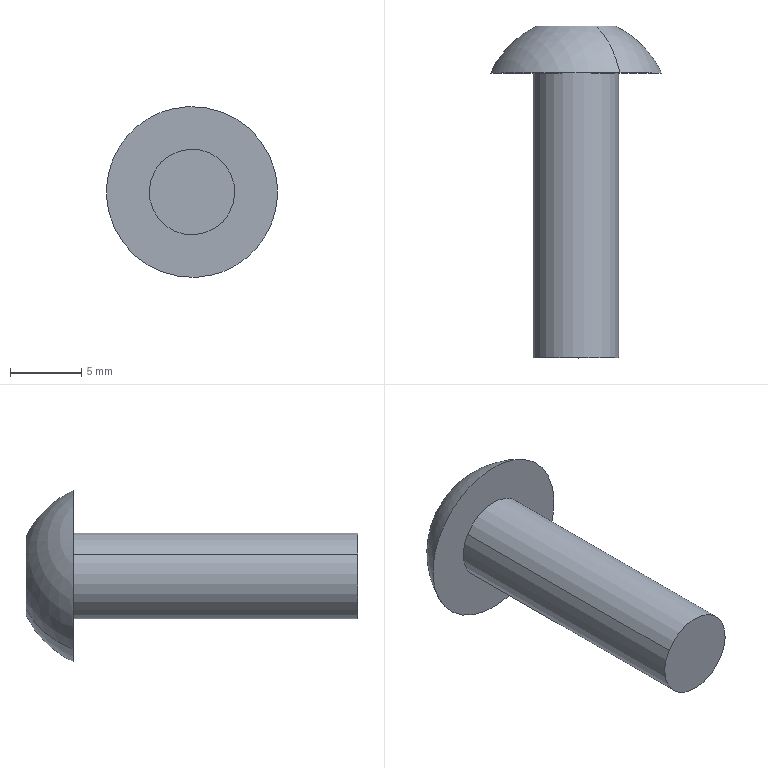Component | SolidWorks | RR40-1_hexagon socket button head screws gb-2 | 1 solid | 19 faces | box 12 x 23.3 x 12 mm | volume 776 mm3 | plane 15 | sphere 2 | cylinder 2 | commonest cylinder face diameters 6 x2
STEP:
#1=COLOUR_RGB('',0.7922,0.8196,0.9333);
#2=FILL_AREA_STYLE_COLOUR('',#1);
#3=FILL_AREA_STYLE('',(#2));
#4=SURFACE_STYLE_FILL_AREA(#3);
#5=SURFACE_SIDE_STYLE('',(#4));
#6=SURFACE_STYLE_USAGE(.BOTH.,#5);
#7=PRESENTATION_STYLE_ASSIGNMENT((#6));
#8=CARTESIAN_POINT('',(23.147,37.717,-81.266));
#9=VERTEX_POINT('',#8);
#10=CARTESIAN_POINT('',(23.39,37.717,-80.861));
#11=VERTEX_POINT('',#10);
#12=CARTESIAN_POINT('',(23.268,37.717,-81.063));
#13=DIRECTION('',(0.,1.,-0.));
#14=DIRECTION('',(0.8574,0.,-0.5146));
#15=AXIS2_PLACEMENT_3D('',#12,#13,#14);
#16=CIRCLE('',#15,0.2362);
#17=EDGE_CURVE('',#9,#11,#16,.T.);
#18=ORIENTED_EDGE('',*,*,#17,.T.);
#19=CARTESIAN_POINT('',(23.324,37.846,-80.97));
#20=VERTEX_POINT('',#19);
#21=CARTESIAN_POINT('',(23.268,37.612,-81.063));
#22=DIRECTION('',(-0.8574,0.,0.5146));
#23=DIRECTION('',(0.5146,0.,0.8574));
#24=AXIS2_PLACEMENT_3D('',#21,#22,#23);
#25=CIRCLE('',#24,0.2584);
#26=EDGE_CURVE('',#11,#20,#25,.T.);
#27=ORIENTED_EDGE('',*,*,#26,.T.);
#28=CARTESIAN_POINT('',(23.213,37.846,-81.156));
#29=VERTEX_POINT('',#28);
#30=CARTESIAN_POINT('',(23.268,37.846,-81.063));
#31=DIRECTION('',(0.,1.,-0.));
#32=DIRECTION('',(0.8574,0.,-0.5146));
#33=AXIS2_PLACEMENT_3D('',#30,#31,#32);
#34=CIRCLE('',#33,0.1083);
#35=EDGE_CURVE('',#29,#20,#34,.T.);
#36=ORIENTED_EDGE('',*,*,#35,.F.);
#37=CARTESIAN_POINT('',(23.268,37.612,-81.063));
#38=DIRECTION('',(0.8574,-0.,-0.5146));
#39=DIRECTION('',(-0.5146,0.,-0.8574));
#40=AXIS2_PLACEMENT_3D('',#37,#38,#39);
#41=CIRCLE('',#40,0.2584);
#42=EDGE_CURVE('',#9,#29,#41,.T.);
#43=ORIENTED_EDGE('',*,*,#42,.F.);
#44=EDGE_LOOP('',(#18,#27,#36,#43));
#45=FACE_OUTER_BOUND('',#44,.T.);
#46=CARTESIAN_POINT('',(23.268,37.612,-81.063));
#47=DIRECTION('',(-0.8574,0.,0.5146));
#48=DIRECTION('',(-0.5146,0.,-0.8574));
#49=AXIS2_PLACEMENT_3D('',#46,#47,#48);
#50=SPHERICAL_SURFACE('',#49,0.2584);
#51=ADVANCED_FACE('',(#45),#50,.T.);
#52=CARTESIAN_POINT('',(23.167,36.929,-81.002));
#53=VERTEX_POINT('',#52);
#54=CARTESIAN_POINT('',(23.37,36.929,-81.124));
#55=VERTEX_POINT('',#54);
#56=CARTESIAN_POINT('',(23.268,36.929,-81.063));
#57=DIRECTION('',(-0.,-1.,0.));
#58=DIRECTION('',(-0.8574,0.,0.5146));
#59=AXIS2_PLACEMENT_3D('',#56,#57,#58);
#60=CIRCLE('',#59,0.1181);
#61=EDGE_CURVE('',#53,#55,#60,.T.);
#62=ORIENTED_EDGE('',*,*,#61,.F.);
#63=CARTESIAN_POINT('',(23.167,37.717,-81.002));
#64=VERTEX_POINT('',#63);
#65=CARTESIAN_POINT('',(23.167,36.929,-81.002));
#66=DIRECTION('',(0.,1.,-0.));
#67=VECTOR('',#66,39.37);
#68=LINE('',#65,#67);
#69=EDGE_CURVE('',#53,#64,#68,.T.);
#70=ORIENTED_EDGE('',*,*,#69,.T.);
#71=CARTESIAN_POINT('',(23.37,37.717,-81.124));
#72=VERTEX_POINT('',#71);
#73=CARTESIAN_POINT('',(23.268,37.717,-81.063));
#74=DIRECTION('',(-0.,-1.,0.));
#75=DIRECTION('',(-0.8574,0.,0.5146));
#76=AXIS2_PLACEMENT_3D('',#73,#74,#75);
#77=CIRCLE('',#76,0.1181);
#78=EDGE_CURVE('',#64,#72,#77,.T.);
#79=ORIENTED_EDGE('',*,*,#78,.T.);
#80=CARTESIAN_POINT('',(23.37,36.929,-81.124));
#81=DIRECTION('',(0.,1.,-0.));
#82=VECTOR('',#81,39.37);
#83=LINE('',#80,#82);
#84=EDGE_CURVE('',#55,#72,#83,.T.);
#85=ORIENTED_EDGE('',*,*,#84,.F.);
#86=EDGE_LOOP('',(#62,#70,#79,#85));
#87=FACE_OUTER_BOUND('',#86,.T.);
#88=CARTESIAN_POINT('',(23.268,36.929,-81.063));
#89=DIRECTION('',(0.,1.,-0.));
#90=DIRECTION('',(0.8574,0.,-0.5146));
#91=AXIS2_PLACEMENT_3D('',#88,#89,#90);
#92=CYLINDRICAL_SURFACE('',#91,0.1181);
#93=ADVANCED_FACE('',(#87),#92,.T.);
#94=ORIENTED_EDGE('',*,*,#35,.T.);
#95=CARTESIAN_POINT('',(23.268,37.846,-81.063));
#96=DIRECTION('',(0.,1.,-0.));
#97=DIRECTION('',(0.8574,0.,-0.5146));
#98=AXIS2_PLACEMENT_3D('',#95,#96,#97);
#99=CIRCLE('',#98,0.1083);
#100=EDGE_CURVE('',#20,#29,#99,.T.);
#101=ORIENTED_EDGE('',*,*,#100,.T.);
#102=EDGE_LOOP('',(#94,#101));
#103=FACE_OUTER_BOUND('',#102,.T.);
#104=CARTESIAN_POINT('',(23.27,37.846,-80.972));
#105=VERTEX_POINT('',#104);
#106=CARTESIAN_POINT('',(23.19,37.846,-81.016));
#107=VERTEX_POINT('',#106);
#108=CARTESIAN_POINT('',(23.27,37.846,-80.972));
#109=DIRECTION('',(-0.8744,0.,-0.4852));
#110=VECTOR('',#109,39.37);
#111=LINE('',#108,#110);
#112=EDGE_CURVE('',#105,#107,#111,.T.);
#113=ORIENTED_EDGE('',*,*,#112,.T.);
#114=CARTESIAN_POINT('',(23.189,37.846,-81.107));
#115=VERTEX_POINT('',#114);
#116=CARTESIAN_POINT('',(23.19,37.846,-81.016));
#117=DIRECTION('',(-0.01698,-0.,-0.9999));
#118=VECTOR('',#117,39.37);
#119=LINE('',#116,#118);
#120=EDGE_CURVE('',#107,#115,#119,.T.);
#121=ORIENTED_EDGE('',*,*,#120,.T.);
#122=CARTESIAN_POINT('',(23.267,37.846,-81.154));
#123=VERTEX_POINT('',#122);
#124=CARTESIAN_POINT('',(23.189,37.846,-81.107));
#125=DIRECTION('',(0.8574,-0.,-0.5146));
#126=VECTOR('',#125,39.37);
#127=LINE('',#124,#126);
#128=EDGE_CURVE('',#115,#123,#127,.T.);
#129=ORIENTED_EDGE('',*,*,#128,.T.);
#130=CARTESIAN_POINT('',(23.346,37.846,-81.11));
#131=VERTEX_POINT('',#130);
#132=CARTESIAN_POINT('',(23.267,37.846,-81.154));
#133=DIRECTION('',(0.8744,-0.,0.4852));
#134=VECTOR('',#133,39.37);
#135=LINE('',#132,#134);
#136=EDGE_CURVE('',#123,#131,#135,.T.);
#137=ORIENTED_EDGE('',*,*,#136,.T.);
#138=CARTESIAN_POINT('',(23.348,37.846,-81.019));
#139=VERTEX_POINT('',#138);
#140=CARTESIAN_POINT('',(23.346,37.846,-81.11));
#141=DIRECTION('',(0.01698,0.,0.9999));
#142=VECTOR('',#141,39.37);
#143=LINE('',#140,#142);
#144=EDGE_CURVE('',#131,#139,#143,.T.);
#145=ORIENTED_EDGE('',*,*,#144,.T.);
#146=CARTESIAN_POINT('',(23.348,37.846,-81.019));
#147=DIRECTION('',(-0.8574,0.,0.5146));
#148=VECTOR('',#147,39.37);
#149=LINE('',#146,#148);
#150=EDGE_CURVE('',#139,#105,#149,.T.);
#151=ORIENTED_EDGE('',*,*,#150,.T.);
#152=EDGE_LOOP('',(#113,#121,#129,#137,#145,#151));
#153=FACE_BOUND('',#152,.T.);
#154=CARTESIAN_POINT('',(23.268,37.846,-81.063));
#155=DIRECTION('',(-0.,-1.,0.));
#156=DIRECTION('',(-0.8574,0.,0.5146));
#157=AXIS2_PLACEMENT_3D('',#154,#155,#156);
#158=PLANE('',#157);
#159=ADVANCED_FACE('',(#103,#153),#158,.F.);
#160=ORIENTED_EDGE('',*,*,#17,.F.);
#161=CARTESIAN_POINT('',(23.268,37.717,-81.063));
#162=DIRECTION('',(0.,1.,-0.));
#163=DIRECTION('',(0.8574,0.,-0.5146));
#164=AXIS2_PLACEMENT_3D('',#161,#162,#163);
#165=CIRCLE('',#164,0.2362);
#166=EDGE_CURVE('',#11,#9,#165,.T.);
#167=ORIENTED_EDGE('',*,*,#166,.F.);
#168=EDGE_LOOP('',(#160,#167));
#169=FACE_OUTER_BOUND('',#168,.T.);
#170=CARTESIAN_POINT('',(23.268,37.717,-81.063));
#171=DIRECTION('',(-0.,-1.,0.));
#172=DIRECTION('',(-0.8574,0.,0.5146));
#173=AXIS2_PLACEMENT_3D('',#170,#171,#172);
#174=CIRCLE('',#173,0.1181);
#175=EDGE_CURVE('',#72,#64,#174,.T.);
#176=ORIENTED_EDGE('',*,*,#175,.F.);
#177=ORIENTED_EDGE('',*,*,#78,.F.);
#178=EDGE_LOOP('',(#176,#177));
#179=FACE_BOUND('',#178,.T.);
#180=CARTESIAN_POINT('',(23.268,37.717,-81.063));
#181=DIRECTION('',(-0.,-1.,0.));
#182=DIRECTION('',(-0.8574,0.,0.5146));
#183=AXIS2_PLACEMENT_3D('',#180,#181,#182);
#184=PLANE('',#183);
#185=ADVANCED_FACE('',(#169,#179),#184,.T.);
#186=ORIENTED_EDGE('',*,*,#69,.F.);
#187=CARTESIAN_POINT('',(23.268,36.929,-81.063));
#188=DIRECTION('',(-0.,-1.,0.));
#189=DIRECTION('',(-0.8574,0.,0.5146));
#190=AXIS2_PLACEMENT_3D('',#187,#188,#189);
#191=CIRCLE('',#190,0.1181);
#192=EDGE_CURVE('',#55,#53,#191,.T.);
#193=ORIENTED_EDGE('',*,*,#192,.F.);
#194=ORIENTED_EDGE('',*,*,#84,.T.);
#195=ORIENTED_EDGE('',*,*,#175,.T.);
#196=EDGE_LOOP('',(#186,#193,#194,#195));
#197=FACE_OUTER_BOUND('',#196,.T.);
#198=CARTESIAN_POINT('',(23.268,36.929,-81.063));
#199=DIRECTION('',(0.,1.,-0.));
#200=DIRECTION('',(0.8574,0.,-0.5146));
#201=AXIS2_PLACEMENT_3D('',#198,#199,#200);
#202=CYLINDRICAL_SURFACE('',#201,0.1181);
#203=ADVANCED_FACE('',(#197),#202,.T.);
#204=ORIENTED_EDGE('',*,*,#192,.T.);
#205=ORIENTED_EDGE('',*,*,#61,.T.);
#206=EDGE_LOOP('',(#204,#205));
#207=FACE_OUTER_BOUND('',#206,.T.);
#208=CARTESIAN_POINT('',(23.268,36.929,-81.063));
#209=DIRECTION('',(-0.,-1.,0.));
#210=DIRECTION('',(-0.8574,0.,0.5146));
#211=AXIS2_PLACEMENT_3D('',#208,#209,#210);
#212=PLANE('',#211);
#213=ADVANCED_FACE('',(#207),#212,.T.);
#214=ORIENTED_EDGE('',*,*,#26,.F.);
#215=ORIENTED_EDGE('',*,*,#166,.T.);
#216=ORIENTED_EDGE('',*,*,#42,.T.);
#217=ORIENTED_EDGE('',*,*,#100,.F.);
#218=EDGE_LOOP('',(#214,#215,#216,#217));
#219=FACE_OUTER_BOUND('',#218,.T.);
#220=CARTESIAN_POINT('',(23.268,37.612,-81.063));
#221=DIRECTION('',(-0.8574,0.,0.5146));
#222=DIRECTION('',(-0.5146,0.,-0.8574));
#223=AXIS2_PLACEMENT_3D('',#220,#221,#222);
#224=SPHERICAL_SURFACE('',#223,0.2584);
#225=ADVANCED_FACE('',(#219),#224,.T.);
#226=ORIENTED_EDGE('',*,*,#112,.F.);
#227=CARTESIAN_POINT('',(23.27,37.765,-80.972));
#228=VERTEX_POINT('',#227);
#229=CARTESIAN_POINT('',(23.27,37.765,-80.972));
#230=DIRECTION('',(0.,1.,-0.));
#231=VECTOR('',#230,39.37);
#232=LINE('',#229,#231);
#233=EDGE_CURVE('',#228,#105,#232,.T.);
#234=ORIENTED_EDGE('',*,*,#233,.F.);
#235=CARTESIAN_POINT('',(23.19,37.765,-81.016));
#236=VERTEX_POINT('',#235);
#237=CARTESIAN_POINT('',(23.27,37.765,-80.972));
#238=DIRECTION('',(-0.8744,0.,-0.4852));
#239=VECTOR('',#238,39.37);
#240=LINE('',#237,#239);
#241=EDGE_CURVE('',#228,#236,#240,.T.);
#242=ORIENTED_EDGE('',*,*,#241,.T.);
#243=CARTESIAN_POINT('',(23.19,37.765,-81.016));
#244=DIRECTION('',(0.,1.,-0.));
#245=VECTOR('',#244,39.37);
#246=LINE('',#243,#245);
#247=EDGE_CURVE('',#236,#107,#246,.T.);
#248=ORIENTED_EDGE('',*,*,#247,.T.);
#249=EDGE_LOOP('',(#226,#234,#242,#248));
#250=FACE_OUTER_BOUND('',#249,.T.);
#251=CARTESIAN_POINT('',(23.27,37.765,-80.972));
#252=DIRECTION('',(0.4852,-0.,-0.8744));
#253=DIRECTION('',(0.8744,-0.,0.4852));
#254=AXIS2_PLACEMENT_3D('',#251,#252,#253);
#255=PLANE('',#254);
#256=ADVANCED_FACE('',(#250),#255,.T.);
#257=ORIENTED_EDGE('',*,*,#120,.F.);
#258=ORIENTED_EDGE('',*,*,#247,.F.);
#259=CARTESIAN_POINT('',(23.189,37.765,-81.107));
#260=VERTEX_POINT('',#259);
#261=CARTESIAN_POINT('',(23.19,37.765,-81.016));
#262=DIRECTION('',(-0.01698,-0.,-0.9999));
#263=VECTOR('',#262,39.37);
#264=LINE('',#261,#263);
#265=EDGE_CURVE('',#236,#260,#264,.T.);
#266=ORIENTED_EDGE('',*,*,#265,.T.);
#267=CARTESIAN_POINT('',(23.189,37.765,-81.107));
#268=DIRECTION('',(0.,1.,-0.));
#269=VECTOR('',#268,39.37);
#270=LINE('',#267,#269);
#271=EDGE_CURVE('',#260,#115,#270,.T.);
#272=ORIENTED_EDGE('',*,*,#271,.T.);
#273=EDGE_LOOP('',(#257,#258,#266,#272));
#274=FACE_OUTER_BOUND('',#273,.T.);
#275=CARTESIAN_POINT('',(23.19,37.765,-81.016));
#276=DIRECTION('',(0.9999,-0.,-0.01698));
#277=DIRECTION('',(0.01698,0.,0.9999));
#278=AXIS2_PLACEMENT_3D('',#275,#276,#277);
#279=PLANE('',#278);
#280=ADVANCED_FACE('',(#274),#279,.T.);
#281=ORIENTED_EDGE('',*,*,#128,.F.);
#282=ORIENTED_EDGE('',*,*,#271,.F.);
#283=CARTESIAN_POINT('',(23.267,37.765,-81.154));
#284=VERTEX_POINT('',#283);
#285=CARTESIAN_POINT('',(23.189,37.765,-81.107));
#286=DIRECTION('',(0.8574,-0.,-0.5146));
#287=VECTOR('',#286,39.37);
#288=LINE('',#285,#287);
#289=EDGE_CURVE('',#260,#284,#288,.T.);
#290=ORIENTED_EDGE('',*,*,#289,.T.);
#291=CARTESIAN_POINT('',(23.267,37.765,-81.154));
#292=DIRECTION('',(0.,1.,-0.));
#293=VECTOR('',#292,39.37);
#294=LINE('',#291,#293);
#295=EDGE_CURVE('',#284,#123,#294,.T.);
#296=ORIENTED_EDGE('',*,*,#295,.T.);
#297=EDGE_LOOP('',(#281,#282,#290,#296));
#298=FACE_OUTER_BOUND('',#297,.T.);
#299=CARTESIAN_POINT('',(23.189,37.765,-81.107));
#300=DIRECTION('',(0.5146,-0.,0.8574));
#301=DIRECTION('',(-0.8574,0.,0.5146));
#302=AXIS2_PLACEMENT_3D('',#299,#300,#301);
#303=PLANE('',#302);
#304=ADVANCED_FACE('',(#298),#303,.T.);
#305=ORIENTED_EDGE('',*,*,#136,.F.);
#306=ORIENTED_EDGE('',*,*,#295,.F.);
#307=CARTESIAN_POINT('',(23.346,37.765,-81.11));
#308=VERTEX_POINT('',#307);
#309=CARTESIAN_POINT('',(23.267,37.765,-81.154));
#310=DIRECTION('',(0.8744,-0.,0.4852));
#311=VECTOR('',#310,39.37);
#312=LINE('',#309,#311);
#313=EDGE_CURVE('',#284,#308,#312,.T.);
#314=ORIENTED_EDGE('',*,*,#313,.T.);
#315=CARTESIAN_POINT('',(23.346,37.765,-81.11));
#316=DIRECTION('',(0.,1.,-0.));
#317=VECTOR('',#316,39.37);
#318=LINE('',#315,#317);
#319=EDGE_CURVE('',#308,#131,#318,.T.);
#320=ORIENTED_EDGE('',*,*,#319,.T.);
#321=EDGE_LOOP('',(#305,#306,#314,#320));
#322=FACE_OUTER_BOUND('',#321,.T.);
#323=CARTESIAN_POINT('',(23.267,37.765,-81.154));
#324=DIRECTION('',(-0.4852,0.,0.8744));
#325=DIRECTION('',(-0.8744,0.,-0.4852));
#326=AXIS2_PLACEMENT_3D('',#323,#324,#325);
#327=PLANE('',#326);
#328=ADVANCED_FACE('',(#322),#327,.T.);
#329=ORIENTED_EDGE('',*,*,#144,.F.);
#330=ORIENTED_EDGE('',*,*,#319,.F.);
#331=CARTESIAN_POINT('',(23.348,37.765,-81.019));
#332=VERTEX_POINT('',#331);
#333=CARTESIAN_POINT('',(23.346,37.765,-81.11));
#334=DIRECTION('',(0.01698,0.,0.9999));
#335=VECTOR('',#334,39.37);
#336=LINE('',#333,#335);
#337=EDGE_CURVE('',#308,#332,#336,.T.);
#338=ORIENTED_EDGE('',*,*,#337,.T.);
#339=CARTESIAN_POINT('',(23.348,37.765,-81.019));
#340=DIRECTION('',(0.,1.,-0.));
#341=VECTOR('',#340,39.37);
#342=LINE('',#339,#341);
#343=EDGE_CURVE('',#332,#139,#342,.T.);
#344=ORIENTED_EDGE('',*,*,#343,.T.);
#345=EDGE_LOOP('',(#329,#330,#338,#344));
#346=FACE_OUTER_BOUND('',#345,.T.);
#347=CARTESIAN_POINT('',(23.346,37.765,-81.11));
#348=DIRECTION('',(-0.9999,0.,0.01698));
#349=DIRECTION('',(-0.01698,-0.,-0.9999));
#350=AXIS2_PLACEMENT_3D('',#347,#348,#349);
#351=PLANE('',#350);
#352=ADVANCED_FACE('',(#346),#351,.T.);
#353=ORIENTED_EDGE('',*,*,#150,.F.);
#354=ORIENTED_EDGE('',*,*,#343,.F.);
#355=CARTESIAN_POINT('',(23.348,37.765,-81.019));
#356=DIRECTION('',(-0.8574,0.,0.5146));
#357=VECTOR('',#356,39.37);
#358=LINE('',#355,#357);
#359=EDGE_CURVE('',#332,#228,#358,.T.);
#360=ORIENTED_EDGE('',*,*,#359,.T.);
#361=ORIENTED_EDGE('',*,*,#233,.T.);
#362=EDGE_LOOP('',(#353,#354,#360,#361));
#363=FACE_OUTER_BOUND('',#362,.T.);
#364=CARTESIAN_POINT('',(23.348,37.765,-81.019));
#365=DIRECTION('',(-0.5146,0.,-0.8574));
#366=DIRECTION('',(0.8574,-0.,-0.5146));
#367=AXIS2_PLACEMENT_3D('',#364,#365,#366);
#368=PLANE('',#367);
#369=ADVANCED_FACE('',(#363),#368,.T.);
#370=ORIENTED_EDGE('',*,*,#337,.F.);
#371=CARTESIAN_POINT('',(23.268,37.719,-81.063));
#372=VERTEX_POINT('',#371);
#373=CARTESIAN_POINT('',(23.346,37.765,-81.11));
#374=DIRECTION('',(0.7669,0.4472,-0.4603));
#375=VECTOR('',#374,39.37);
#376=LINE('',#373,#375);
#377=EDGE_CURVE('',#372,#308,#376,.T.);
#378=ORIENTED_EDGE('',*,*,#377,.F.);
#379=CARTESIAN_POINT('',(23.348,37.765,-81.019));
#380=DIRECTION('',(0.7821,0.4472,0.434));
#381=VECTOR('',#380,39.37);
#382=LINE('',#379,#381);
#383=EDGE_CURVE('',#372,#332,#382,.T.);
#384=ORIENTED_EDGE('',*,*,#383,.T.);
#385=EDGE_LOOP('',(#370,#378,#384));
#386=FACE_OUTER_BOUND('',#385,.T.);
#387=CARTESIAN_POINT('',(23.346,37.765,-81.11));
#388=DIRECTION('',(0.4999,-0.866,-0.008488));
#389=DIRECTION('',(-0.7669,-0.4472,0.4603));
#390=AXIS2_PLACEMENT_3D('',#387,#388,#389);
#391=PLANE('',#390);
#392=ADVANCED_FACE('',(#386),#391,.F.);
#393=ORIENTED_EDGE('',*,*,#359,.F.);
#394=ORIENTED_EDGE('',*,*,#383,.F.);
#395=CARTESIAN_POINT('',(23.27,37.765,-80.972));
#396=DIRECTION('',(0.01518,0.4472,0.8943));
#397=VECTOR('',#396,39.37);
#398=LINE('',#395,#397);
#399=EDGE_CURVE('',#372,#228,#398,.T.);
#400=ORIENTED_EDGE('',*,*,#399,.T.);
#401=EDGE_LOOP('',(#393,#394,#400));
#402=FACE_OUTER_BOUND('',#401,.T.);
#403=CARTESIAN_POINT('',(23.348,37.765,-81.019));
#404=DIRECTION('',(0.2573,-0.866,0.4287));
#405=DIRECTION('',(-0.4457,-0.5,-0.7425));
#406=AXIS2_PLACEMENT_3D('',#403,#404,#405);
#407=PLANE('',#406);
#408=ADVANCED_FACE('',(#402),#407,.F.);
#409=ORIENTED_EDGE('',*,*,#241,.F.);
#410=ORIENTED_EDGE('',*,*,#399,.F.);
#411=CARTESIAN_POINT('',(23.19,37.765,-81.016));
#412=DIRECTION('',(-0.7669,0.4472,0.4603));
#413=VECTOR('',#412,39.37);
#414=LINE('',#411,#413);
#415=EDGE_CURVE('',#372,#236,#414,.T.);
#416=ORIENTED_EDGE('',*,*,#415,.T.);
#417=EDGE_LOOP('',(#409,#410,#416));
#418=FACE_OUTER_BOUND('',#417,.T.);
#419=CARTESIAN_POINT('',(23.27,37.765,-80.972));
#420=DIRECTION('',(-0.2426,-0.866,0.4372));
#421=DIRECTION('',(-0.7669,0.4472,0.4603));
#422=AXIS2_PLACEMENT_3D('',#419,#420,#421);
#423=PLANE('',#422);
#424=ADVANCED_FACE('',(#418),#423,.F.);
#425=ORIENTED_EDGE('',*,*,#265,.F.);
#426=ORIENTED_EDGE('',*,*,#415,.F.);
#427=CARTESIAN_POINT('',(23.189,37.765,-81.107));
#428=DIRECTION('',(-0.7821,0.4472,-0.434));
#429=VECTOR('',#428,39.37);
#430=LINE('',#427,#429);
#431=EDGE_CURVE('',#372,#260,#430,.T.);
#432=ORIENTED_EDGE('',*,*,#431,.T.);
#433=EDGE_LOOP('',(#425,#426,#432));
#434=FACE_OUTER_BOUND('',#433,.T.);
#435=CARTESIAN_POINT('',(23.19,37.765,-81.016));
#436=DIRECTION('',(-0.4999,-0.866,0.008488));
#437=DIRECTION('',(-0.7669,0.4472,0.4603));
#438=AXIS2_PLACEMENT_3D('',#435,#436,#437);
#439=PLANE('',#438);
#440=ADVANCED_FACE('',(#434),#439,.F.);
#441=ORIENTED_EDGE('',*,*,#289,.F.);
#442=ORIENTED_EDGE('',*,*,#431,.F.);
#443=CARTESIAN_POINT('',(23.267,37.765,-81.154));
#444=DIRECTION('',(-0.01518,0.4472,-0.8943));
#445=VECTOR('',#444,39.37);
#446=LINE('',#443,#445);
#447=EDGE_CURVE('',#372,#284,#446,.T.);
#448=ORIENTED_EDGE('',*,*,#447,.T.);
#449=EDGE_LOOP('',(#441,#442,#448));
#450=FACE_OUTER_BOUND('',#449,.T.);
#451=CARTESIAN_POINT('',(23.189,37.765,-81.107));
#452=DIRECTION('',(-0.2573,-0.866,-0.4287));
#453=DIRECTION('',(-0.4457,0.5,-0.7425));
#454=AXIS2_PLACEMENT_3D('',#451,#452,#453);
#455=PLANE('',#454);
#456=ADVANCED_FACE('',(#450),#455,.F.);
#457=ORIENTED_EDGE('',*,*,#313,.F.);
#458=ORIENTED_EDGE('',*,*,#447,.F.);
#459=ORIENTED_EDGE('',*,*,#377,.T.);
#460=EDGE_LOOP('',(#457,#458,#459));
#461=FACE_OUTER_BOUND('',#460,.T.);
#462=CARTESIAN_POINT('',(23.267,37.765,-81.154));
#463=DIRECTION('',(0.2426,-0.866,-0.4372));
#464=DIRECTION('',(-0.7669,-0.4472,0.4603));
#465=AXIS2_PLACEMENT_3D('',#462,#463,#464);
#466=PLANE('',#465);
#467=ADVANCED_FACE('',(#461),#466,.F.);
#468=CLOSED_SHELL('',(#51,#93,#159,#185,#203,#213,#225,#256,#280,#304,#328,#352,#369,#392,#408,#424,#440,#456,#467));
#469=MANIFOLD_SOLID_BREP('',#468);
#470=STYLED_ITEM('',(#7),#469);
#471=(LENGTH_UNIT()NAMED_UNIT(*)SI_UNIT($,.METRE.));
#472=LENGTH_MEASURE_WITH_UNIT(LENGTH_MEASURE(0.0254),#471);
#473=DIMENSIONAL_EXPONENTS(1.,0.,0.,0.,0.,0.,0.);
#474=(CONVERSION_BASED_UNIT('',#472)LENGTH_UNIT()NAMED_UNIT(#473));
#475=UNCERTAINTY_MEASURE_WITH_UNIT(LENGTH_MEASURE(0.00001),#474,'','');
#476=(NAMED_UNIT(*)PLANE_ANGLE_UNIT()SI_UNIT($,.RADIAN.));
#477=(NAMED_UNIT(*)SI_UNIT($,.STERADIAN.)SOLID_ANGLE_UNIT());
#478=(GEOMETRIC_REPRESENTATION_CONTEXT(3)GLOBAL_UNCERTAINTY_ASSIGNED_CONTEXT((#475))GLOBAL_UNIT_ASSIGNED_CONTEXT((#474,#476,#477))REPRESENTATION_CONTEXT('',''));
#479=MECHANICAL_DESIGN_GEOMETRIC_PRESENTATION_REPRESENTATION('',(#470),#478);
#480=PRESENTATION_LAYER_ASSIGNMENT('','',(#470));
#481=CARTESIAN_POINT('',(0.,0.,0.));
#482=DIRECTION('',(0.,0.,1.));
#483=DIRECTION('',(1.,0.,0.));
#484=AXIS2_PLACEMENT_3D('',#481,#482,#483);
#485=(LENGTH_UNIT()NAMED_UNIT(*)SI_UNIT($,.METRE.));
#486=LENGTH_MEASURE_WITH_UNIT(LENGTH_MEASURE(0.0254),#485);
#487=DIMENSIONAL_EXPONENTS(1.,0.,0.,0.,0.,0.,0.);
#488=(CONVERSION_BASED_UNIT('',#486)LENGTH_UNIT()NAMED_UNIT(#487));
#489=UNCERTAINTY_MEASURE_WITH_UNIT(LENGTH_MEASURE(0.00001),#488,'','');
#490=(NAMED_UNIT(*)PLANE_ANGLE_UNIT()SI_UNIT($,.RADIAN.));
#491=(NAMED_UNIT(*)SI_UNIT($,.STERADIAN.)SOLID_ANGLE_UNIT());
#492=(GEOMETRIC_REPRESENTATION_CONTEXT(3)GLOBAL_UNCERTAINTY_ASSIGNED_CONTEXT((#489))GLOBAL_UNIT_ASSIGNED_CONTEXT((#488,#490,#491))REPRESENTATION_CONTEXT('',''));
#493=ADVANCED_BREP_SHAPE_REPRESENTATION('',(#469,#484),#492);